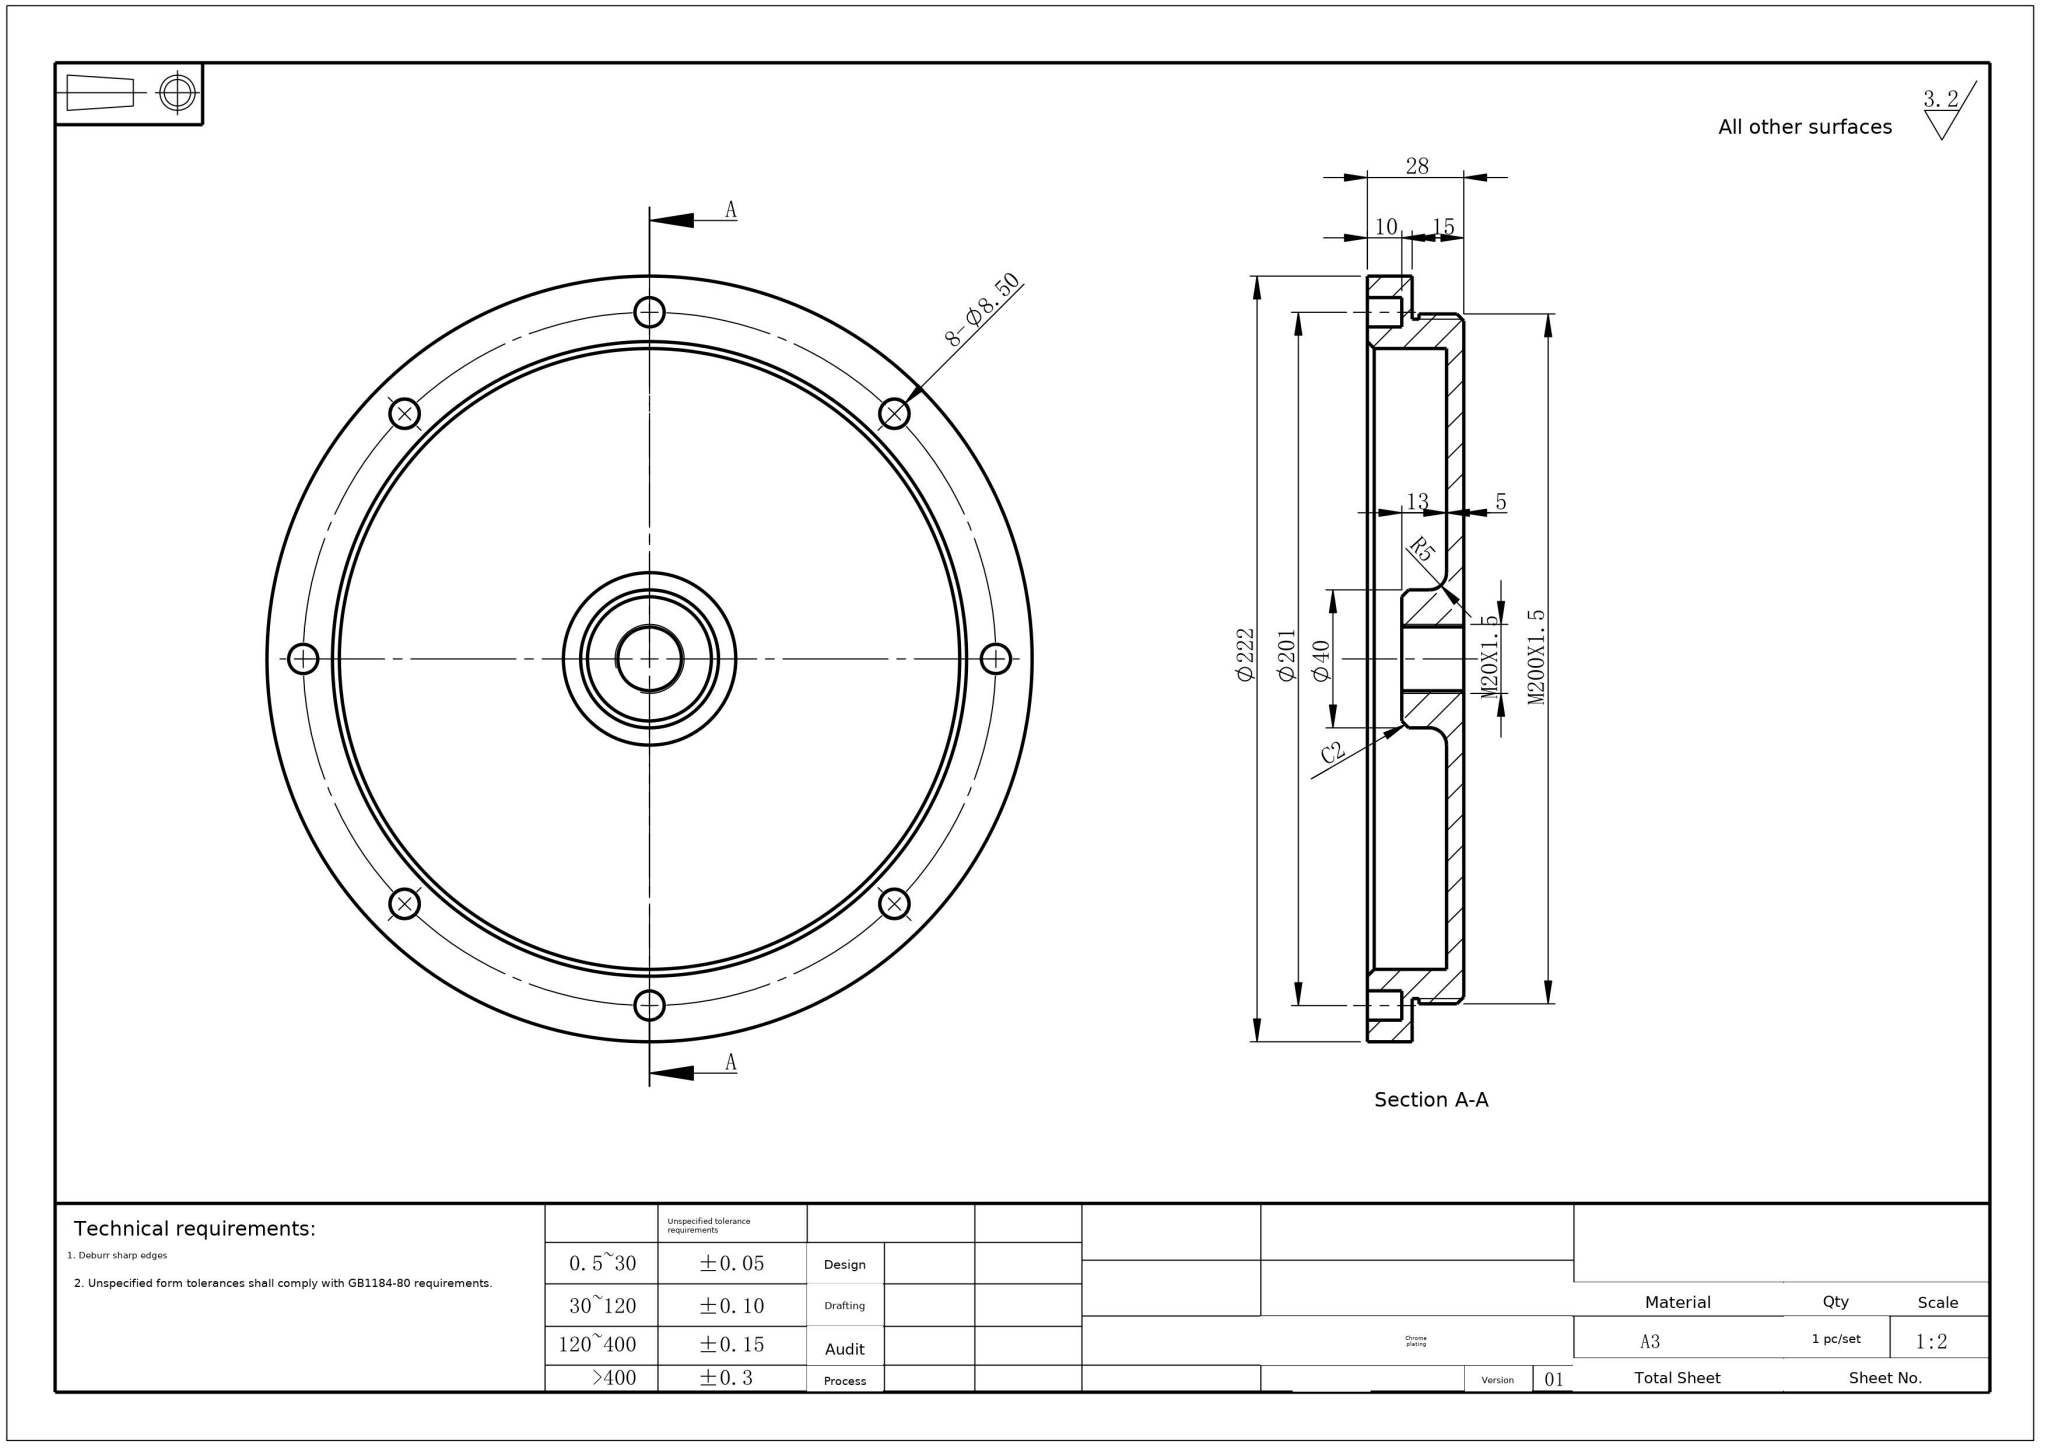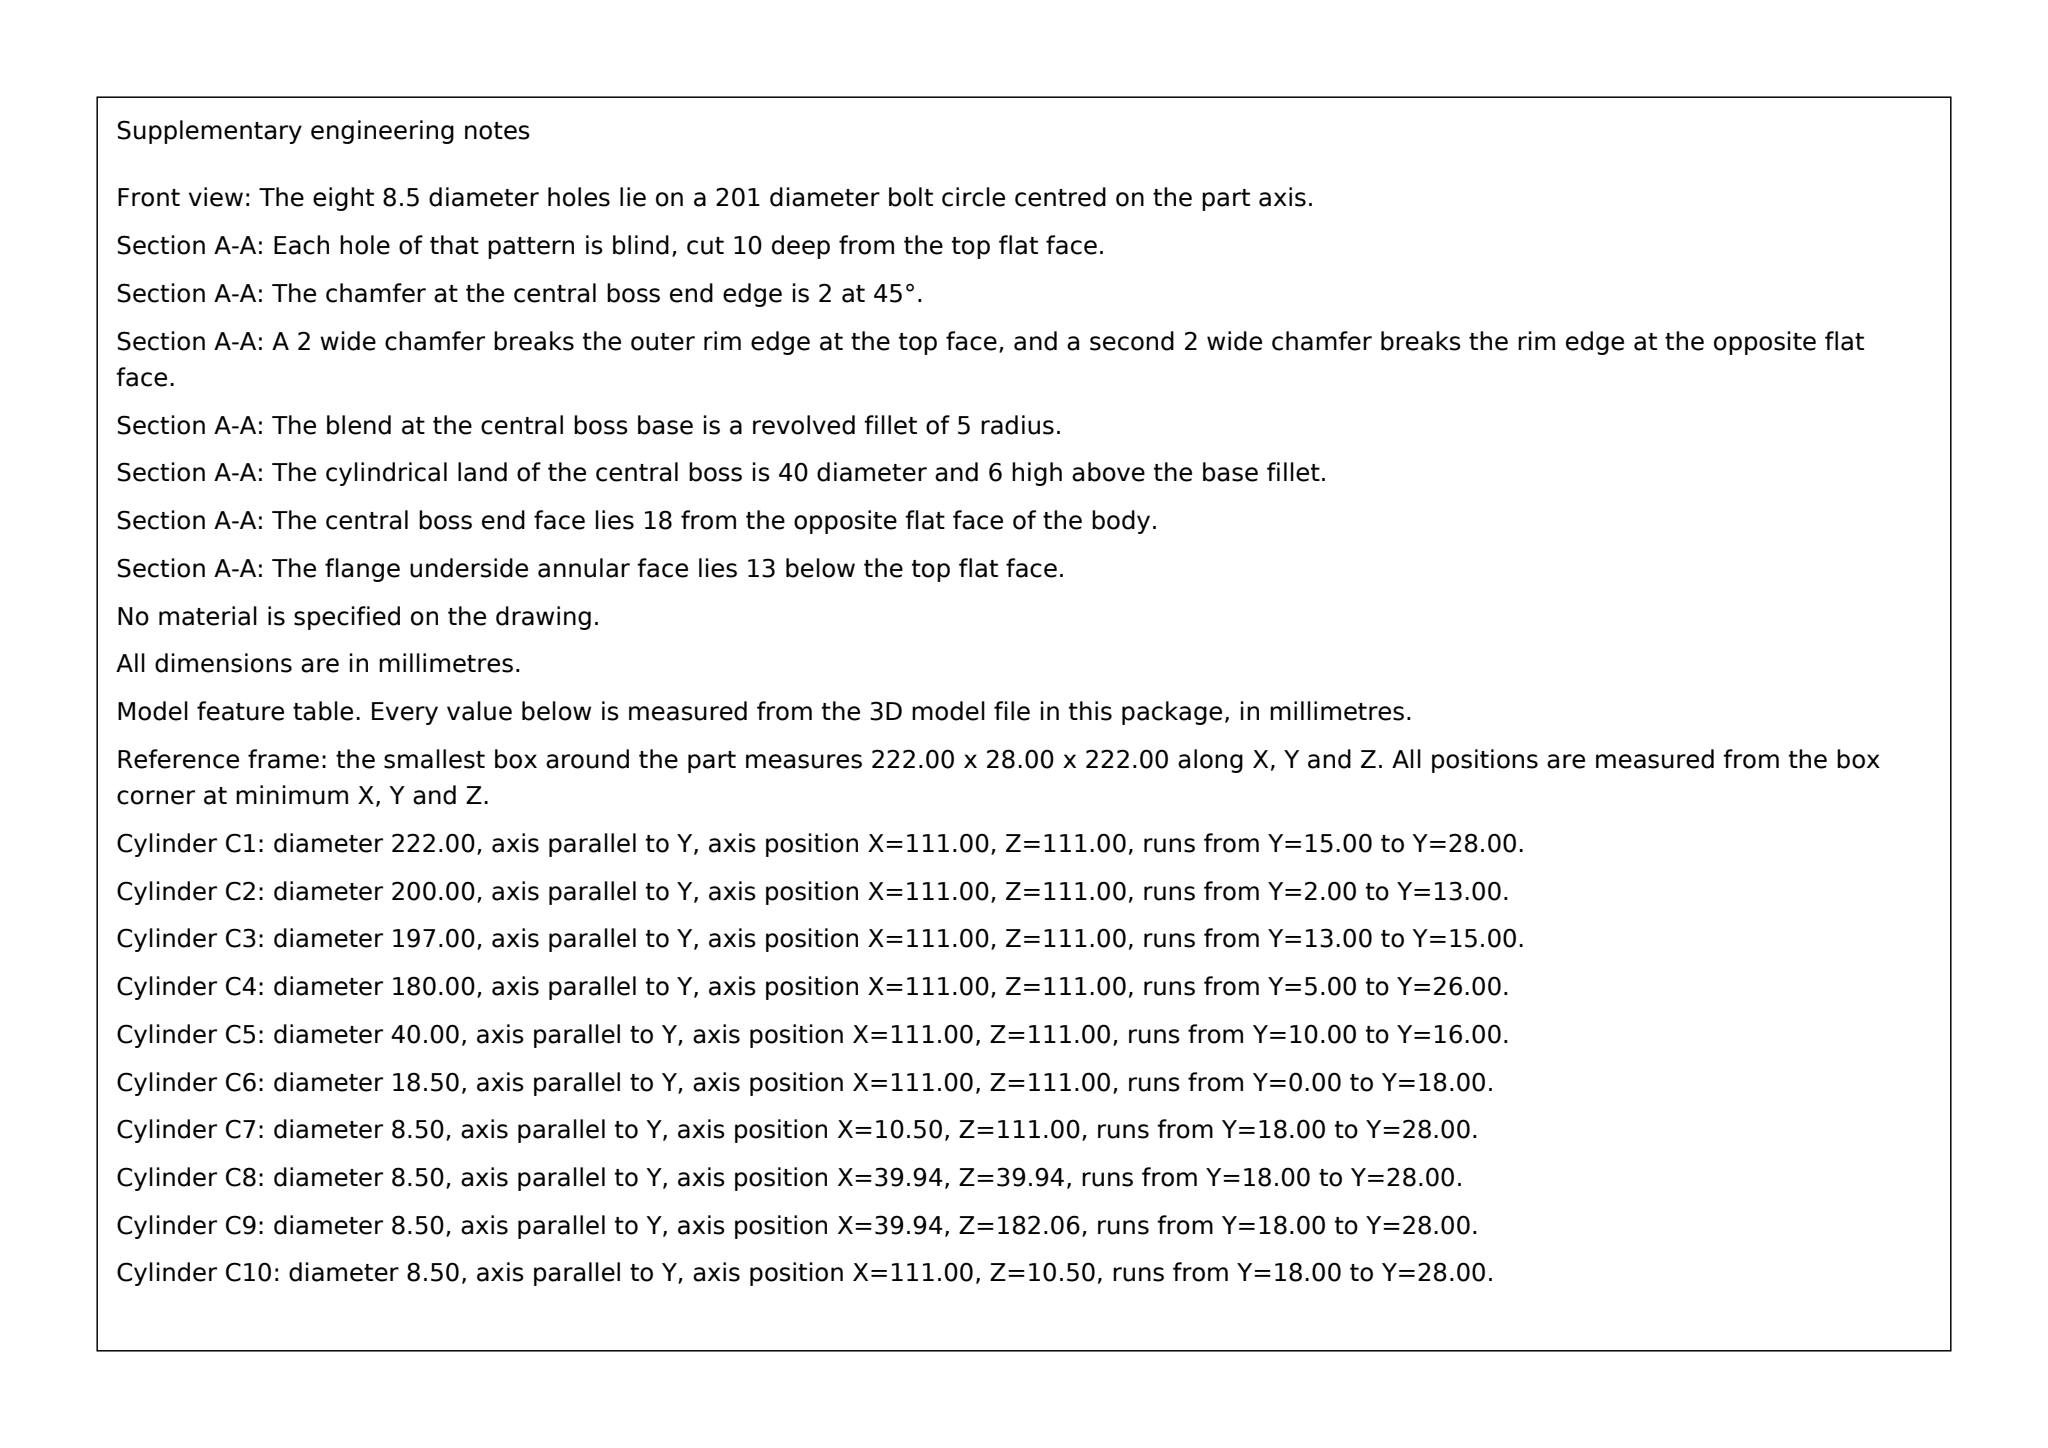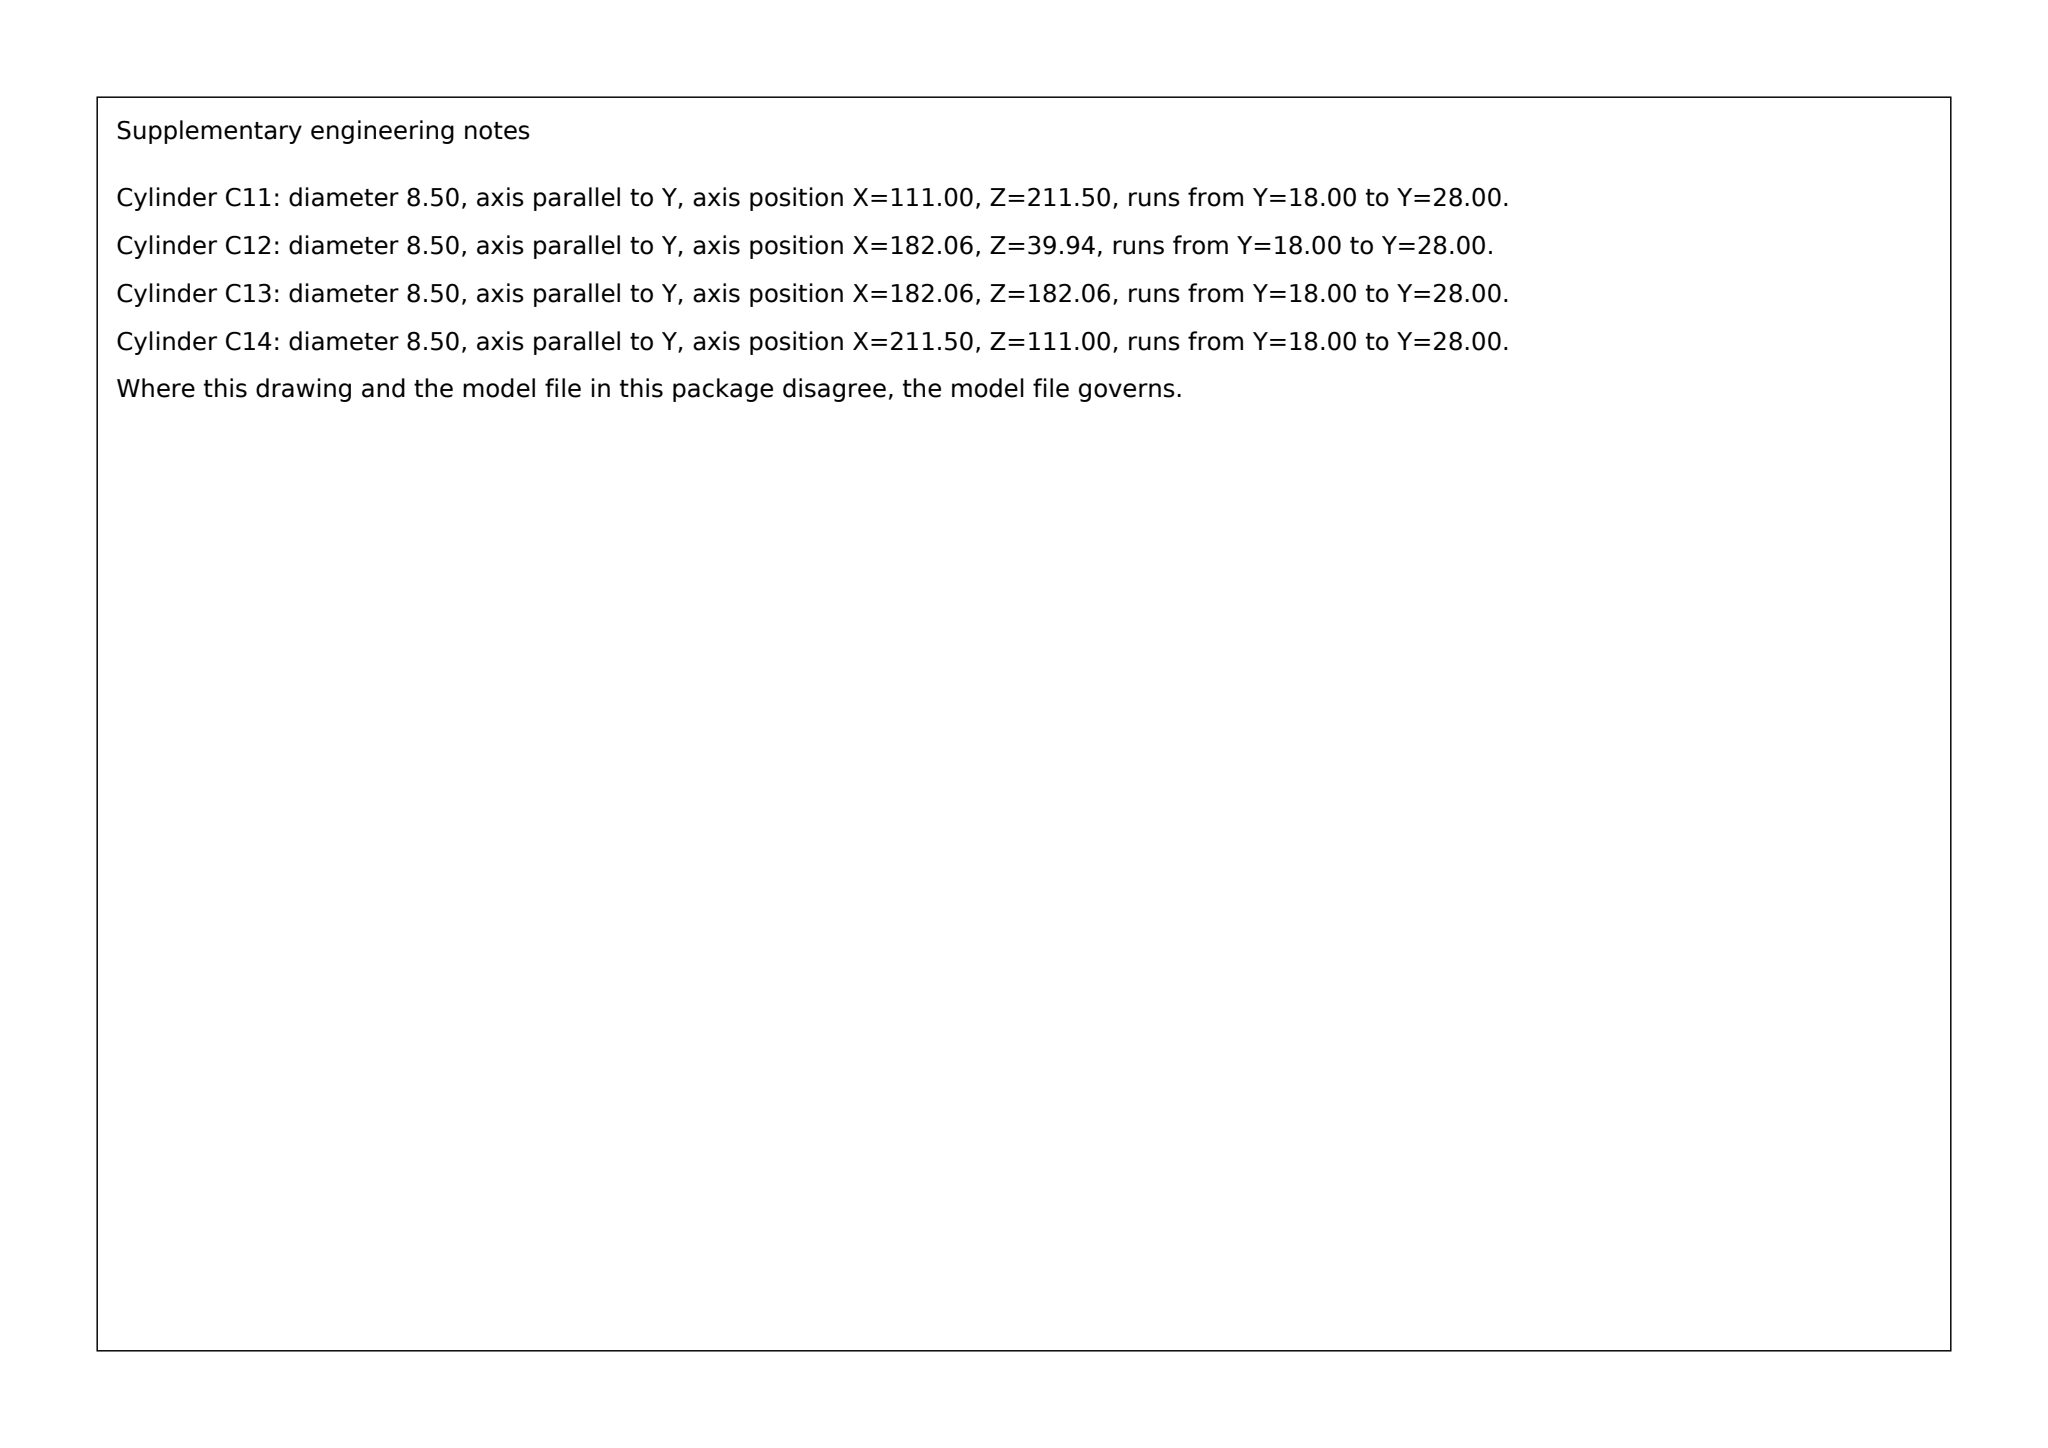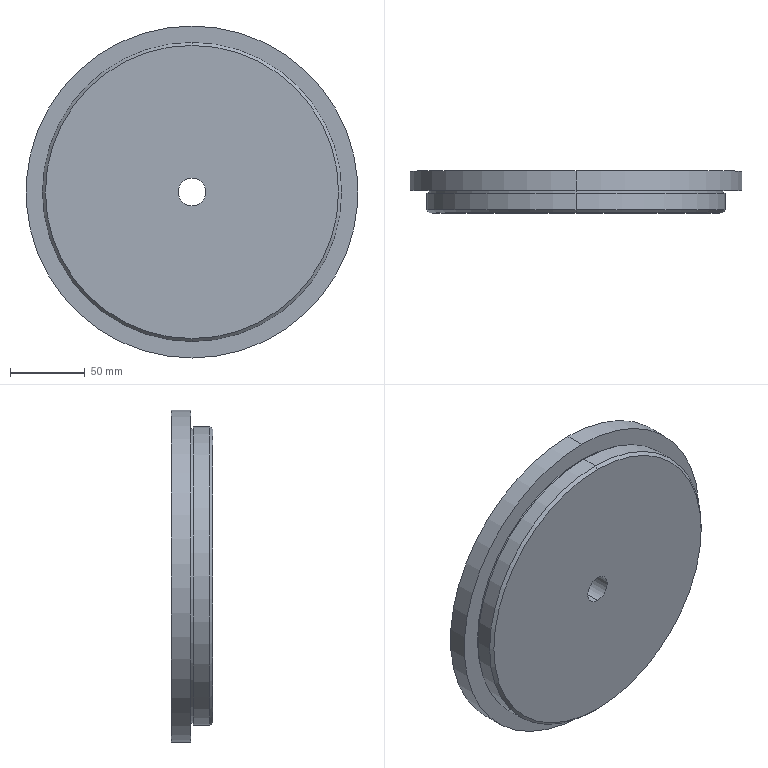Part | SolidWorks | mm | 1 solid | 50 faces | box 222 x 28 x 222 mm | volume 392327 mm3 | cylinder 28 | plane 14 | cone 6 | torus 2 | commonest cylinder face diameters 8.5 x16 18.5 x2 200 x2 197 x2 222 x2 180 x2 40 x2
build123d program:
from build123d import *

# Parameters (mm, degrees)
M20X1_5_TAPPED_HOLE1_D     = 18.5
M20X1_5_TAPPED_HOLE1_DEPTH = 44.5
M20X1_5_TAPPED_HOLE1_TIP   = 5.558
SKETCH4_R                  = 4.25
CUT_EXTRUDE1_DEPTH         = 10
CIRPATTERN1_COUNT          = 8
CHAMFER1_SIZE              = 2


with BuildPart() as part:
    # Sketch1 → Revolve1 (revolve)
    with BuildSketch(Plane.XY, mode=Mode.PRIVATE) as revolve1_sk:
        with BuildLine():
            Line((0, 0), (100, 0))
            Line((100, 0), (100, 13))
            Line((100, 13), (98.5, 13))
            Line((98.5, 13), (98.5, 15))
            Line((98.5, 15), (111, 15))
            Line((111, 15), (111, 28))
            Line((111, 28), (90, 28))
            Line((90, 28), (90, 5))
            Line((90, 5), (25, 5))
            ThreePointArc((25, 5), (21.464, 6.464), (20, 10))
            Line((20, 10), (20, 18))
            Line((20, 18), (0, 18))
            Line((0, 18), (0, 0))
        make_face()
    revolve(revolve1_sk.sketch.rotate(Axis((0, -998.841, 0), (0, 1, 0)), 90), axis=Axis((0, -998.841, 0), (0, 1, 0)))

    # M20x1.5 Tapped Hole1
    with Locations(Plane(origin=(0, 18, 0), x_dir=(-1, 0, 0), z_dir=(0, 1, 0))):
        with Locations((0, 0)):
            Hole(M20X1_5_TAPPED_HOLE1_D / 2, depth=M20X1_5_TAPPED_HOLE1_DEPTH)
            with Locations((0, 0, -(M20X1_5_TAPPED_HOLE1_DEPTH + M20X1_5_TAPPED_HOLE1_TIP / 2))):  # 118° drill point
                Cone(0, M20X1_5_TAPPED_HOLE1_D / 2, M20X1_5_TAPPED_HOLE1_TIP, mode=Mode.SUBTRACT)

    # Sketch4 → Cut-Extrude1 (cut)
    with BuildSketch(Plane(origin=(0, 28, 0), x_dir=(1, 0, 0), z_dir=(0, 1, 0))):
        with Locations(Location((0, -100.5, 0), (0, 0, 270))):
            Circle(SKETCH4_R)
    cut_extrude1 = extrude(amount=-CUT_EXTRUDE1_DEPTH, mode=Mode.SUBTRACT)

    # CirPattern1: Cut-Extrude1 ×8 about axis
    cirpattern1_axis = Axis((0, 0, 0), (0, 1, 0))
    for i in range(1, CIRPATTERN1_COUNT):
        add(cut_extrude1.rotate(cirpattern1_axis, i * 360 / CIRPATTERN1_COUNT), mode=Mode.SUBTRACT)

    # Chamfer1
    chamfer1_edges = [part.edges().sort_by_distance(p)[0] for p in [
        (0, 28, 90),
        (0, 18, 20),
        (0, 0, 100),
    ]]
    chamfer(chamfer1_edges, length=CHAMFER1_SIZE)


solid = part.part